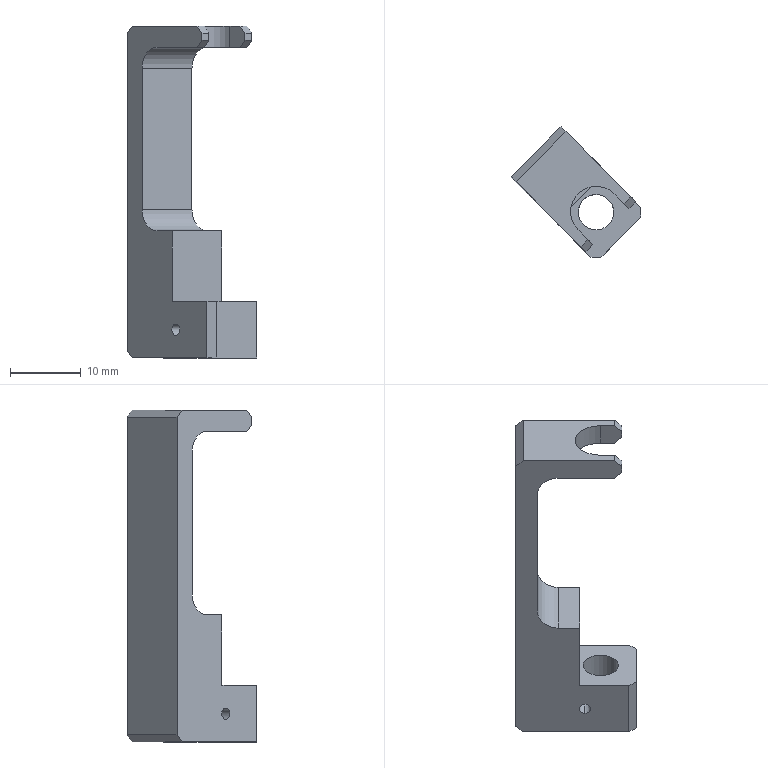Component | SolidWorks | InnerAdjustmentBlock-1 | 1 solid | 34 faces | volume 3197 mm3 | plane 24 | cylinder 10 | commonest cylinder face diameters 1.6 x3 3.3 x2 5 x2 6 x2 7.2 x1